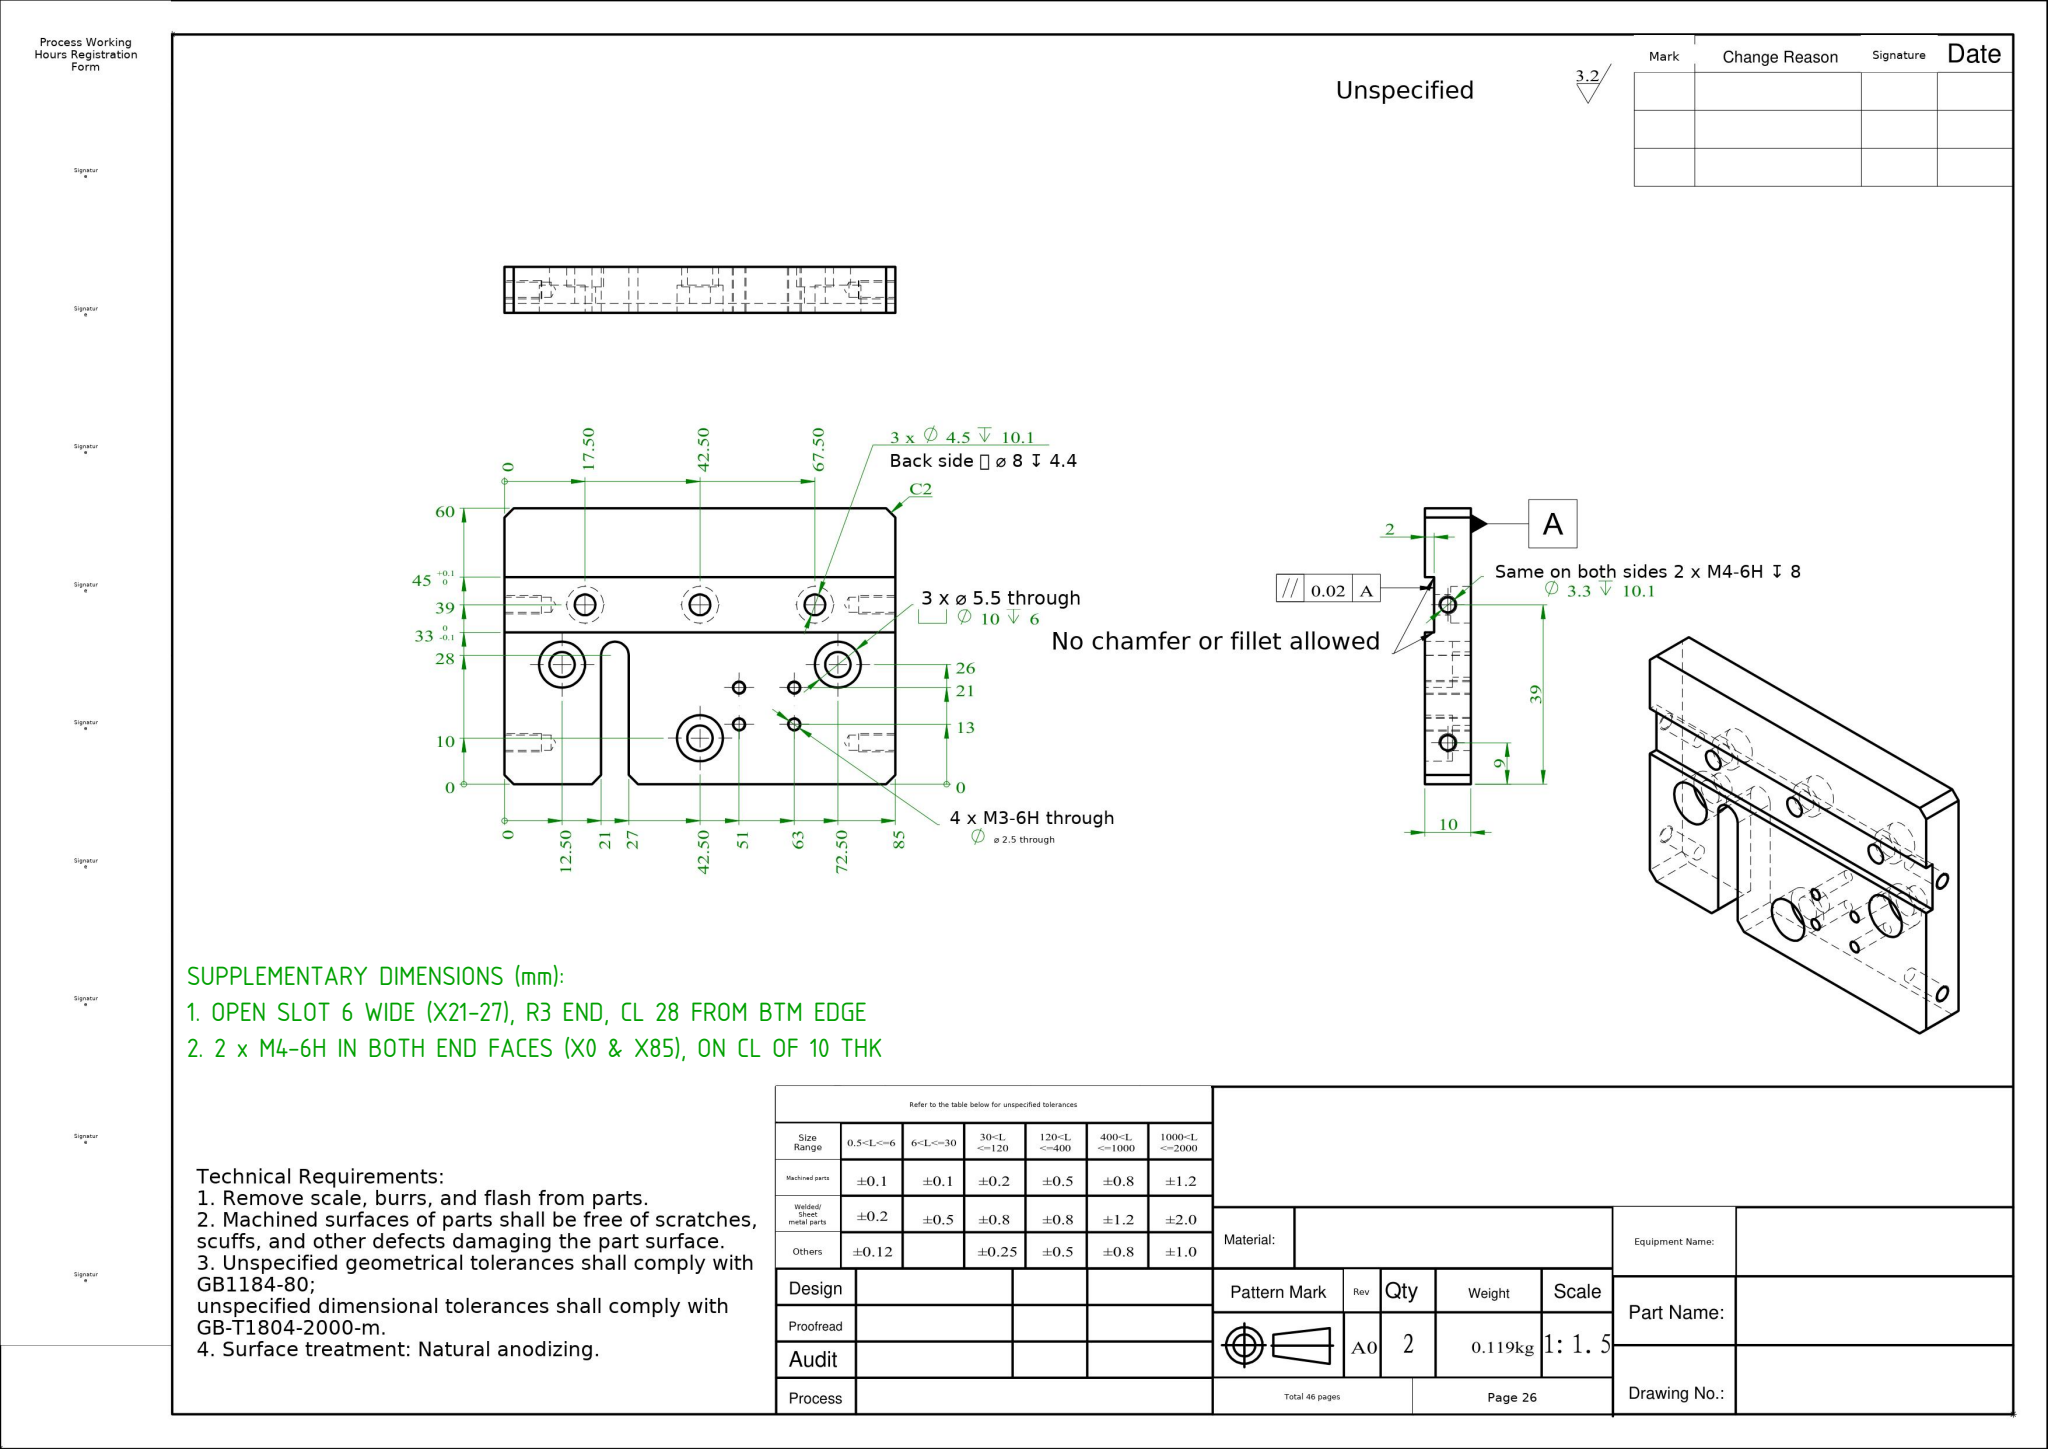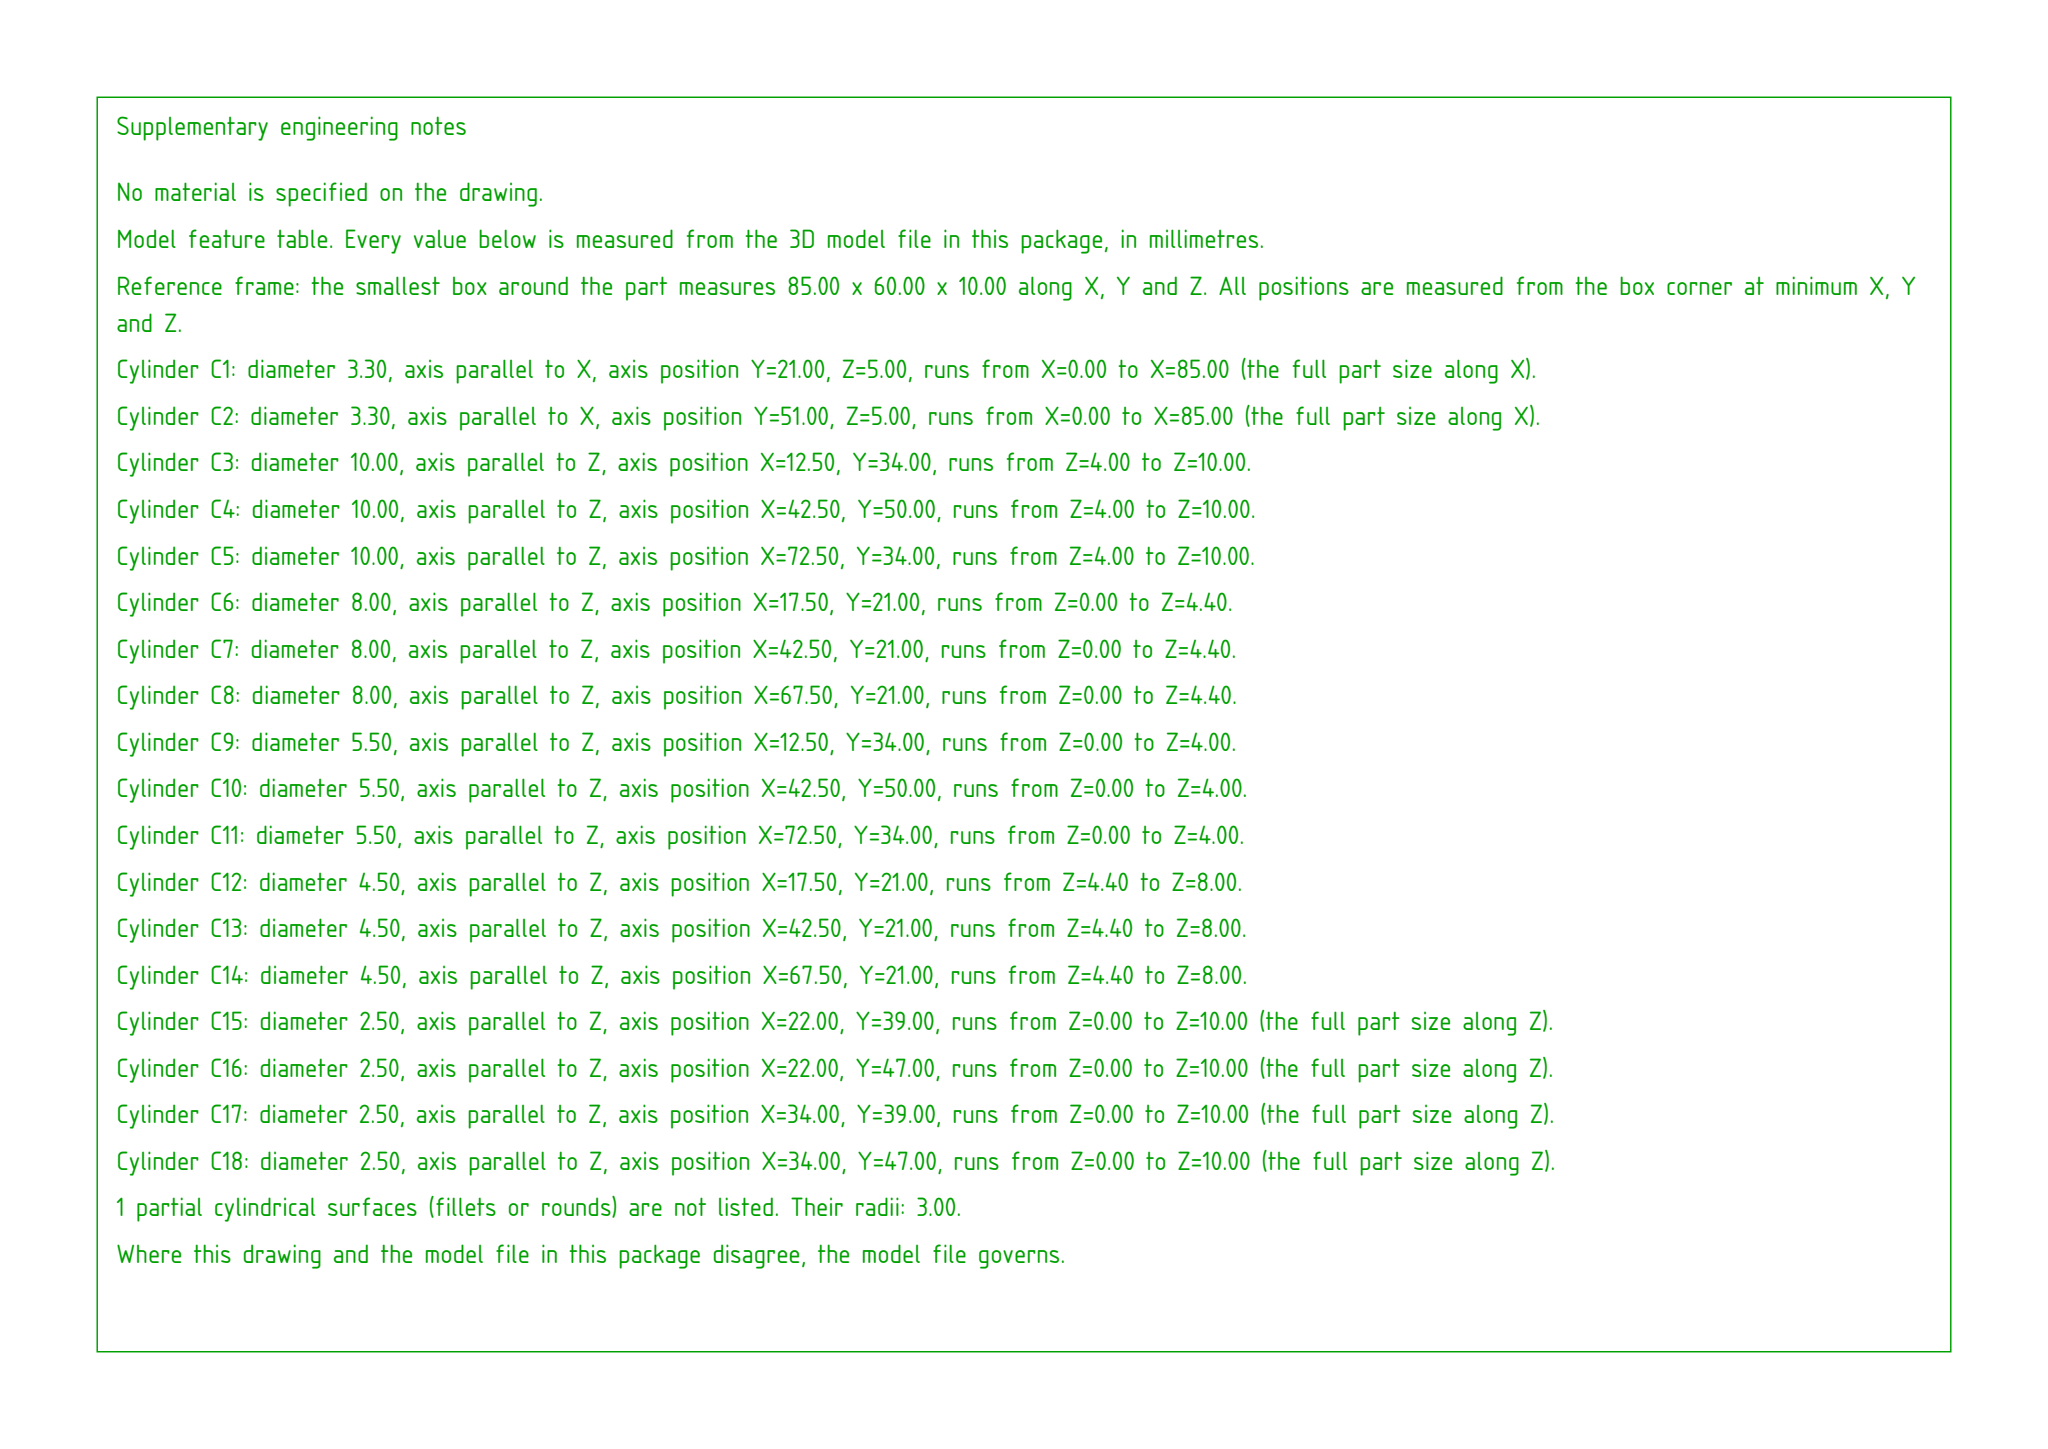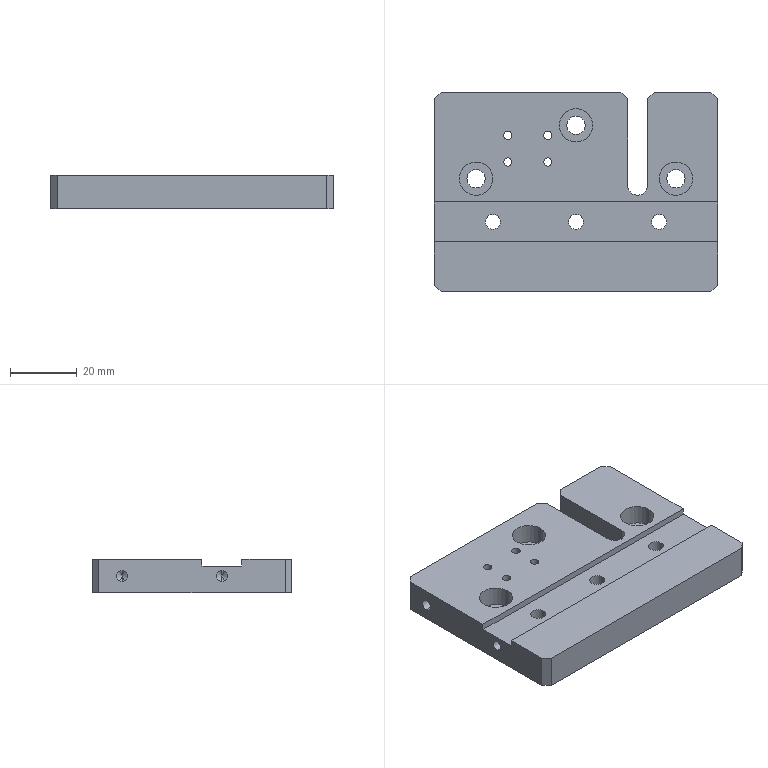Part | SolidWorks | mm | 1 solid | 74 faces | box 85 x 60 x 10 mm | volume 43931 mm3 | cylinder 41 | plane 25 | cone 8 | commonest cylinder face diameters 3.3 x8 2.5 x8 8 x6 4.5 x6 10 x6 5.5 x6 6 x1
build123d program:
from build123d import *

# Parameters (mm, degrees)
SKETCH1_W                                       = 85
SKETCH1_H                                       = 60
BOSS_EXTRUDE1_DEPTH                             = 10
CUT_EXTRUDE1_DEPTH                              = 10
M3_TAPPED_HOLE1_D                               = 2.5
LPATTERN1_COUNT                                 = 2
LPATTERN1_PITCH                                 = 8
M5_HEX_SOCKET_HEAD_CAP_SCREW_CBORE1_D           = 5.5
M5_HEX_SOCKET_HEAD_CAP_SCREW_CBORE1_CBORE_D     = 10
M5_HEX_SOCKET_HEAD_CAP_SCREW_CBORE1_CBORE_DEPTH = 6
M4_TAPPED_HOLE1_AT_2_COUNT                      = 2
M4_TAPPED_HOLE1_AT_2_PITCH                      = 30
M4_HEX_SOCKET_HEAD_CAP_SCREW_CBORE1_D           = 4.5
M4_HEX_SOCKET_HEAD_CAP_SCREW_CBORE1_DEPTH       = 10.1
M4_HEX_SOCKET_HEAD_CAP_SCREW_CBORE1_CBORE_D     = 8
M4_HEX_SOCKET_HEAD_CAP_SCREW_CBORE1_CBORE_DEPTH = 4.4
M4_HEX_SOCKET_HEAD_CAP_SCREW_CBORE1_TIP         = 1.352
CHAMFER1_SIZE                                   = 2
CHAMFER2_SIZE                                   = 2
SKETCH13_W                                      = 3.688
SKETCH13_H                                      = 12
CUT_EXTRUDE3_DEPTH                              = 105.523


with BuildPart() as part:
    # Sketch1 → Boss-Extrude1 (new body)
    with BuildSketch(Plane.XY):
        with Locations((-42.5, 30)):
            Rectangle(SKETCH1_W, SKETCH1_H)
    extrude(amount=BOSS_EXTRUDE1_DEPTH)

    # Sketch2 → Cut-Extrude1 (cut)
    with BuildSketch(Plane(origin=(0, 0, 0), x_dir=(-1, 0, 0), z_dir=(0, 0, -1))):
        with BuildLine():
            Line((21, 32), (21, 65.275))
            ThreePointArc((21, 65.275), (24, 68.275), (27, 65.275))
            Line((27, 65.275), (27, 32))
            ThreePointArc((27, 32), (24, 29), (21, 32))
        make_face()
    extrude(amount=-CUT_EXTRUDE1_DEPTH, mode=Mode.SUBTRACT)

    # M3 Tapped Hole1 (through all)
    with Locations(Plane.XY.offset(10)):
        with Locations((-51, 47), (-63, 47)):
            m3_tapped_hole1 = Hole(M3_TAPPED_HOLE1_D / 2)

    # LPattern1: M3 Tapped Hole1 ×2
    with Locations(*[(0, -i * LPATTERN1_PITCH, 0) for i in range(1, LPATTERN1_COUNT)]):
        add(m3_tapped_hole1, mode=Mode.SUBTRACT)

    # M5 Hex Socket Head Cap Screw CBORE1 (through all)
    with Locations(Plane.XY.offset(10)):
        with Locations((-72.5, 34), (-12.5, 34), (-42.5, 50)):
            CounterBoreHole(M5_HEX_SOCKET_HEAD_CAP_SCREW_CBORE1_D / 2, M5_HEX_SOCKET_HEAD_CAP_SCREW_CBORE1_CBORE_D / 2, M5_HEX_SOCKET_HEAD_CAP_SCREW_CBORE1_CBORE_DEPTH)

    # Sketch9 → M4 Tapped Hole1 (revolve, cut)
    with BuildSketch(Plane(origin=(0, 21, 5), x_dir=(0, 0, -1), z_dir=(0, 1, 0))):
        Polygon((0, 0), (0, 11.091), (1.65, 10.1), (1.65, 0), align=None)
    m4_tapped_hole1 = revolve(axis=Axis((6.35, 21, 5), (-1, 0, 0)), mode=Mode.SUBTRACT)

    # M4 Tapped Hole1 at 2: M4 Tapped Hole1 ×2
    with Locations(*[(0, i * M4_TAPPED_HOLE1_AT_2_PITCH, 0) for i in range(1, M4_TAPPED_HOLE1_AT_2_COUNT)]):
        add(m4_tapped_hole1, mode=Mode.SUBTRACT)

    # M4 Hex Socket Head Cap Screw CBORE1
    with Locations(Plane(origin=(0, 0, 0), x_dir=(-1, 0, 0), z_dir=(0, 0, -1))):
        with Locations((17.5, 21), (42.5, 21), (67.5, 21)):
            CounterBoreHole(M4_HEX_SOCKET_HEAD_CAP_SCREW_CBORE1_D / 2, M4_HEX_SOCKET_HEAD_CAP_SCREW_CBORE1_CBORE_D / 2, M4_HEX_SOCKET_HEAD_CAP_SCREW_CBORE1_CBORE_DEPTH, depth=M4_HEX_SOCKET_HEAD_CAP_SCREW_CBORE1_DEPTH)
            with Locations((0, 0, -(M4_HEX_SOCKET_HEAD_CAP_SCREW_CBORE1_DEPTH + M4_HEX_SOCKET_HEAD_CAP_SCREW_CBORE1_TIP / 2))):  # 118° drill point
                Cone(0, M4_HEX_SOCKET_HEAD_CAP_SCREW_CBORE1_D / 2, M4_HEX_SOCKET_HEAD_CAP_SCREW_CBORE1_TIP, mode=Mode.SUBTRACT)

    # Mirror1: M4 Tapped Hole1 across plane
    add(m4_tapped_hole1.mirror(Plane.ZY.offset(42.5)), mode=Mode.SUBTRACT)

    # Mirror1 copy 1 sketch → Mirror1 copy 1 (revolve, cut)
    with BuildSketch(Plane(origin=(-85, 51, 5), x_dir=(0, 0, -1), z_dir=(0, 1, 0))):
        Polygon((0, 0), (0, -11.091), (1.65, -10.1), (1.65, 0), align=None)
    revolve(axis=Axis((-91.35, 51, 5), (-1, 0, 0)), mode=Mode.SUBTRACT)

    # Chamfer1
    chamfer1_edges = [part.edges().sort_by_distance(p)[0] for p in [
        (0, 0, 5),
        (-85, 0, 5),
        (-85, 60, 5),
        (0, 60, 5),
    ]]
    chamfer(chamfer1_edges, length=CHAMFER1_SIZE)

    # Chamfer2
    chamfer2_edges = [part.edges().sort_by_distance(p)[0] for p in [
        (-21, 60, 5),
        (-27, 60, 5),
    ]]
    chamfer(chamfer2_edges, length=CHAMFER2_SIZE)

    # Sketch13 → Cut-Extrude3 (cut, through all)
    with BuildSketch(Plane.ZY.offset(85)):
        with Locations((9.844, 21)):
            Rectangle(SKETCH13_W, SKETCH13_H)
    extrude(amount=-CUT_EXTRUDE3_DEPTH, mode=Mode.SUBTRACT)


solid = part.part